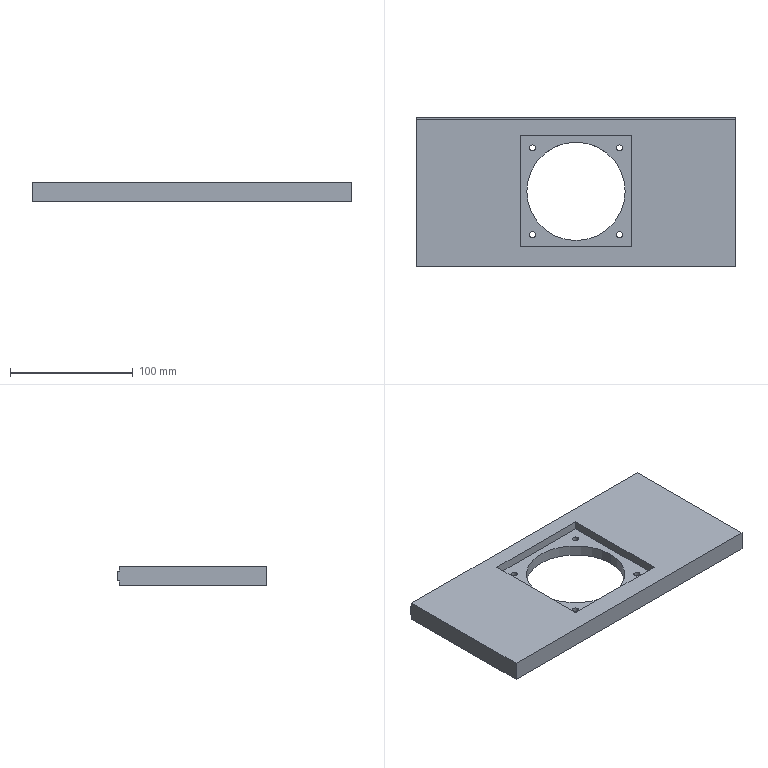Component | SolidWorks | NewTypeCurveBenderReducerPlate-DoubleWheel-2_NewTypeCurveBenderReducerPlate-DoubleWheel-1 | 1 solid | 25 faces | box 260 x 122 x 16 mm | volume 400082 mm3 | plane 15 | cylinder 10 | commonest cylinder face diameters 5 x8 80 x2
STEP:
#1=CARTESIAN_POINT('',(1.49,-3.38,7.559));
#2=VERTEX_POINT('',#1);
#3=CARTESIAN_POINT('',(1.294,-3.38,7.559));
#4=VERTEX_POINT('',#3);
#5=CARTESIAN_POINT('',(1.392,-3.38,7.559));
#6=DIRECTION('',(-0.,-0.,1.));
#7=DIRECTION('',(-1.,0.,0.));
#8=AXIS2_PLACEMENT_3D('',#5,#6,#7);
#9=CIRCLE('',#8,0.09843);
#10=EDGE_CURVE('',#2,#4,#9,.T.);
#11=ORIENTED_EDGE('',*,*,#10,.F.);
#12=CARTESIAN_POINT('',(1.49,-3.38,7.913));
#13=VERTEX_POINT('',#12);
#14=CARTESIAN_POINT('',(1.49,-3.38,8.031));
#15=DIRECTION('',(-0.,-0.,1.));
#16=VECTOR('',#15,39.37);
#17=LINE('',#14,#16);
#18=EDGE_CURVE('',#2,#13,#17,.T.);
#19=ORIENTED_EDGE('',*,*,#18,.T.);
#20=CARTESIAN_POINT('',(1.294,-3.38,7.913));
#21=VERTEX_POINT('',#20);
#22=CARTESIAN_POINT('',(1.392,-3.38,7.913));
#23=DIRECTION('',(-0.,-0.,1.));
#24=DIRECTION('',(1.,0.,0.));
#25=AXIS2_PLACEMENT_3D('',#22,#23,#24);
#26=CIRCLE('',#25,0.09843);
#27=EDGE_CURVE('',#13,#21,#26,.T.);
#28=ORIENTED_EDGE('',*,*,#27,.T.);
#29=CARTESIAN_POINT('',(1.294,-3.38,8.031));
#30=DIRECTION('',(-0.,-0.,1.));
#31=VECTOR('',#30,39.37);
#32=LINE('',#29,#31);
#33=EDGE_CURVE('',#4,#21,#32,.T.);
#34=ORIENTED_EDGE('',*,*,#33,.F.);
#35=EDGE_LOOP('',(#11,#19,#28,#34));
#36=FACE_OUTER_BOUND('',#35,.T.);
#37=CARTESIAN_POINT('',(1.392,-3.38,8.031));
#38=DIRECTION('',(-0.,-0.,1.));
#39=DIRECTION('',(-1.,0.,0.));
#40=AXIS2_PLACEMENT_3D('',#37,#38,#39);
#41=CYLINDRICAL_SURFACE('',#40,0.09843);
#42=ADVANCED_FACE('',(#36),#41,.F.);
#43=CARTESIAN_POINT('',(-1.294,-3.38,7.559));
#44=VERTEX_POINT('',#43);
#45=CARTESIAN_POINT('',(-1.49,-3.38,7.559));
#46=VERTEX_POINT('',#45);
#47=CARTESIAN_POINT('',(-1.392,-3.38,7.559));
#48=DIRECTION('',(-0.,-0.,1.));
#49=DIRECTION('',(-1.,0.,0.));
#50=AXIS2_PLACEMENT_3D('',#47,#48,#49);
#51=CIRCLE('',#50,0.09843);
#52=EDGE_CURVE('',#44,#46,#51,.T.);
#53=ORIENTED_EDGE('',*,*,#52,.F.);
#54=CARTESIAN_POINT('',(-1.294,-3.38,7.913));
#55=VERTEX_POINT('',#54);
#56=CARTESIAN_POINT('',(-1.294,-3.38,8.031));
#57=DIRECTION('',(-0.,-0.,1.));
#58=VECTOR('',#57,39.37);
#59=LINE('',#56,#58);
#60=EDGE_CURVE('',#44,#55,#59,.T.);
#61=ORIENTED_EDGE('',*,*,#60,.T.);
#62=CARTESIAN_POINT('',(-1.49,-3.38,7.913));
#63=VERTEX_POINT('',#62);
#64=CARTESIAN_POINT('',(-1.392,-3.38,7.913));
#65=DIRECTION('',(-0.,-0.,1.));
#66=DIRECTION('',(1.,0.,0.));
#67=AXIS2_PLACEMENT_3D('',#64,#65,#66);
#68=CIRCLE('',#67,0.09843);
#69=EDGE_CURVE('',#55,#63,#68,.T.);
#70=ORIENTED_EDGE('',*,*,#69,.T.);
#71=CARTESIAN_POINT('',(-1.49,-3.38,8.031));
#72=DIRECTION('',(-0.,-0.,1.));
#73=VECTOR('',#72,39.37);
#74=LINE('',#71,#73);
#75=EDGE_CURVE('',#46,#63,#74,.T.);
#76=ORIENTED_EDGE('',*,*,#75,.F.);
#77=EDGE_LOOP('',(#53,#61,#70,#76));
#78=FACE_OUTER_BOUND('',#77,.T.);
#79=CARTESIAN_POINT('',(-1.392,-3.38,8.031));
#80=DIRECTION('',(-0.,-0.,1.));
#81=DIRECTION('',(-1.,0.,0.));
#82=AXIS2_PLACEMENT_3D('',#79,#80,#81);
#83=CYLINDRICAL_SURFACE('',#82,0.09843);
#84=ADVANCED_FACE('',(#78),#83,.F.);
#85=CARTESIAN_POINT('',(-1.294,-0.5962,7.559));
#86=VERTEX_POINT('',#85);
#87=CARTESIAN_POINT('',(-1.49,-0.5962,7.559));
#88=VERTEX_POINT('',#87);
#89=CARTESIAN_POINT('',(-1.392,-0.5962,7.559));
#90=DIRECTION('',(-0.,-0.,1.));
#91=DIRECTION('',(-1.,0.,0.));
#92=AXIS2_PLACEMENT_3D('',#89,#90,#91);
#93=CIRCLE('',#92,0.09843);
#94=EDGE_CURVE('',#86,#88,#93,.T.);
#95=ORIENTED_EDGE('',*,*,#94,.F.);
#96=CARTESIAN_POINT('',(-1.294,-0.5962,7.913));
#97=VERTEX_POINT('',#96);
#98=CARTESIAN_POINT('',(-1.294,-0.5962,8.031));
#99=DIRECTION('',(-0.,-0.,1.));
#100=VECTOR('',#99,39.37);
#101=LINE('',#98,#100);
#102=EDGE_CURVE('',#86,#97,#101,.T.);
#103=ORIENTED_EDGE('',*,*,#102,.T.);
#104=CARTESIAN_POINT('',(-1.49,-0.5962,7.913));
#105=VERTEX_POINT('',#104);
#106=CARTESIAN_POINT('',(-1.392,-0.5962,7.913));
#107=DIRECTION('',(-0.,-0.,1.));
#108=DIRECTION('',(1.,0.,0.));
#109=AXIS2_PLACEMENT_3D('',#106,#107,#108);
#110=CIRCLE('',#109,0.09843);
#111=EDGE_CURVE('',#97,#105,#110,.T.);
#112=ORIENTED_EDGE('',*,*,#111,.T.);
#113=CARTESIAN_POINT('',(-1.49,-0.5962,8.031));
#114=DIRECTION('',(-0.,-0.,1.));
#115=VECTOR('',#114,39.37);
#116=LINE('',#113,#115);
#117=EDGE_CURVE('',#88,#105,#116,.T.);
#118=ORIENTED_EDGE('',*,*,#117,.F.);
#119=EDGE_LOOP('',(#95,#103,#112,#118));
#120=FACE_OUTER_BOUND('',#119,.T.);
#121=CARTESIAN_POINT('',(-1.392,-0.5962,8.031));
#122=DIRECTION('',(-0.,-0.,1.));
#123=DIRECTION('',(-1.,0.,0.));
#124=AXIS2_PLACEMENT_3D('',#121,#122,#123);
#125=CYLINDRICAL_SURFACE('',#124,0.09843);
#126=ADVANCED_FACE('',(#120),#125,.F.);
#127=CARTESIAN_POINT('',(1.49,-0.5962,7.559));
#128=VERTEX_POINT('',#127);
#129=CARTESIAN_POINT('',(1.294,-0.5962,7.559));
#130=VERTEX_POINT('',#129);
#131=CARTESIAN_POINT('',(1.392,-0.5962,7.559));
#132=DIRECTION('',(-0.,-0.,1.));
#133=DIRECTION('',(-1.,0.,0.));
#134=AXIS2_PLACEMENT_3D('',#131,#132,#133);
#135=CIRCLE('',#134,0.09843);
#136=EDGE_CURVE('',#128,#130,#135,.T.);
#137=ORIENTED_EDGE('',*,*,#136,.F.);
#138=CARTESIAN_POINT('',(1.49,-0.5962,7.913));
#139=VERTEX_POINT('',#138);
#140=CARTESIAN_POINT('',(1.49,-0.5962,8.031));
#141=DIRECTION('',(-0.,-0.,1.));
#142=VECTOR('',#141,39.37);
#143=LINE('',#140,#142);
#144=EDGE_CURVE('',#128,#139,#143,.T.);
#145=ORIENTED_EDGE('',*,*,#144,.T.);
#146=CARTESIAN_POINT('',(1.294,-0.5962,7.913));
#147=VERTEX_POINT('',#146);
#148=CARTESIAN_POINT('',(1.392,-0.5962,7.913));
#149=DIRECTION('',(-0.,-0.,1.));
#150=DIRECTION('',(1.,0.,0.));
#151=AXIS2_PLACEMENT_3D('',#148,#149,#150);
#152=CIRCLE('',#151,0.09843);
#153=EDGE_CURVE('',#139,#147,#152,.T.);
#154=ORIENTED_EDGE('',*,*,#153,.T.);
#155=CARTESIAN_POINT('',(1.294,-0.5962,8.031));
#156=DIRECTION('',(-0.,-0.,1.));
#157=VECTOR('',#156,39.37);
#158=LINE('',#155,#157);
#159=EDGE_CURVE('',#130,#147,#158,.T.);
#160=ORIENTED_EDGE('',*,*,#159,.F.);
#161=EDGE_LOOP('',(#137,#145,#154,#160));
#162=FACE_OUTER_BOUND('',#161,.T.);
#163=CARTESIAN_POINT('',(1.392,-0.5962,8.031));
#164=DIRECTION('',(-0.,-0.,1.));
#165=DIRECTION('',(-1.,0.,0.));
#166=AXIS2_PLACEMENT_3D('',#163,#164,#165);
#167=CYLINDRICAL_SURFACE('',#166,0.09843);
#168=ADVANCED_FACE('',(#162),#167,.F.);
#169=CARTESIAN_POINT('',(1.575,-1.988,7.559));
#170=VERTEX_POINT('',#169);
#171=CARTESIAN_POINT('',(-1.575,-1.988,7.559));
#172=VERTEX_POINT('',#171);
#173=CARTESIAN_POINT('',(0.,-1.988,7.559));
#174=DIRECTION('',(-0.,-0.,1.));
#175=DIRECTION('',(-1.,0.,0.));
#176=AXIS2_PLACEMENT_3D('',#173,#174,#175);
#177=CIRCLE('',#176,1.575);
#178=EDGE_CURVE('',#170,#172,#177,.T.);
#179=ORIENTED_EDGE('',*,*,#178,.F.);
#180=CARTESIAN_POINT('',(1.575,-1.988,7.913));
#181=VERTEX_POINT('',#180);
#182=CARTESIAN_POINT('',(1.575,-1.988,7.402));
#183=DIRECTION('',(-0.,-0.,1.));
#184=VECTOR('',#183,39.37);
#185=LINE('',#182,#184);
#186=EDGE_CURVE('',#170,#181,#185,.T.);
#187=ORIENTED_EDGE('',*,*,#186,.T.);
#188=CARTESIAN_POINT('',(-1.575,-1.988,7.913));
#189=VERTEX_POINT('',#188);
#190=CARTESIAN_POINT('',(0.,-1.988,7.913));
#191=DIRECTION('',(-0.,-0.,1.));
#192=DIRECTION('',(1.,0.,0.));
#193=AXIS2_PLACEMENT_3D('',#190,#191,#192);
#194=CIRCLE('',#193,1.575);
#195=EDGE_CURVE('',#181,#189,#194,.T.);
#196=ORIENTED_EDGE('',*,*,#195,.T.);
#197=CARTESIAN_POINT('',(-1.575,-1.988,7.402));
#198=DIRECTION('',(-0.,-0.,1.));
#199=VECTOR('',#198,39.37);
#200=LINE('',#197,#199);
#201=EDGE_CURVE('',#172,#189,#200,.T.);
#202=ORIENTED_EDGE('',*,*,#201,.F.);
#203=EDGE_LOOP('',(#179,#187,#196,#202));
#204=FACE_OUTER_BOUND('',#203,.T.);
#205=CARTESIAN_POINT('',(0.,-1.988,7.402));
#206=DIRECTION('',(-0.,-0.,1.));
#207=DIRECTION('',(-1.,0.,0.));
#208=AXIS2_PLACEMENT_3D('',#205,#206,#207);
#209=CYLINDRICAL_SURFACE('',#208,1.575);
#210=ADVANCED_FACE('',(#204),#209,.F.);
#211=CARTESIAN_POINT('',(-5.118,0.315,8.031));
#212=VERTEX_POINT('',#211);
#213=CARTESIAN_POINT('',(5.118,0.315,8.031));
#214=VERTEX_POINT('',#213);
#215=CARTESIAN_POINT('',(-5.118,0.315,8.031));
#216=DIRECTION('',(1.,-0.,0.));
#217=VECTOR('',#216,39.37);
#218=LINE('',#215,#217);
#219=EDGE_CURVE('',#212,#214,#218,.T.);
#220=ORIENTED_EDGE('',*,*,#219,.F.);
#221=CARTESIAN_POINT('',(-5.118,0.315,8.189));
#222=VERTEX_POINT('',#221);
#223=CARTESIAN_POINT('',(-5.118,0.315,8.189));
#224=DIRECTION('',(0.,0.,-1.));
#225=VECTOR('',#224,39.37);
#226=LINE('',#223,#225);
#227=EDGE_CURVE('',#222,#212,#226,.T.);
#228=ORIENTED_EDGE('',*,*,#227,.F.);
#229=CARTESIAN_POINT('',(5.118,0.315,8.189));
#230=VERTEX_POINT('',#229);
#231=CARTESIAN_POINT('',(5.118,0.315,8.189));
#232=DIRECTION('',(-1.,0.,-0.));
#233=VECTOR('',#232,39.37);
#234=LINE('',#231,#233);
#235=EDGE_CURVE('',#230,#222,#234,.T.);
#236=ORIENTED_EDGE('',*,*,#235,.F.);
#237=CARTESIAN_POINT('',(5.118,0.315,8.189));
#238=DIRECTION('',(0.,0.,-1.));
#239=VECTOR('',#238,39.37);
#240=LINE('',#237,#239);
#241=EDGE_CURVE('',#230,#214,#240,.T.);
#242=ORIENTED_EDGE('',*,*,#241,.T.);
#243=EDGE_LOOP('',(#220,#228,#236,#242));
#244=FACE_OUTER_BOUND('',#243,.T.);
#245=CARTESIAN_POINT('',(5.118,0.315,8.189));
#246=DIRECTION('',(-0.,-1.,-0.));
#247=DIRECTION('',(-0.,-0.,1.));
#248=AXIS2_PLACEMENT_3D('',#245,#246,#247);
#249=PLANE('',#248);
#250=ADVANCED_FACE('',(#244),#249,.F.);
#251=CARTESIAN_POINT('',(-5.118,0.315,7.559));
#252=VERTEX_POINT('',#251);
#253=CARTESIAN_POINT('',(-5.118,-4.409,7.559));
#254=VERTEX_POINT('',#253);
#255=CARTESIAN_POINT('',(-5.118,-4.409,7.559));
#256=DIRECTION('',(0.,-1.,-0.));
#257=VECTOR('',#256,39.37);
#258=LINE('',#255,#257);
#259=EDGE_CURVE('',#252,#254,#258,.T.);
#260=ORIENTED_EDGE('',*,*,#259,.T.);
#261=CARTESIAN_POINT('',(-5.118,-4.409,8.189));
#262=VERTEX_POINT('',#261);
#263=CARTESIAN_POINT('',(-5.118,-4.409,8.189));
#264=DIRECTION('',(0.,0.,-1.));
#265=VECTOR('',#264,39.37);
#266=LINE('',#263,#265);
#267=EDGE_CURVE('',#262,#254,#266,.T.);
#268=ORIENTED_EDGE('',*,*,#267,.F.);
#269=CARTESIAN_POINT('',(-5.118,-4.409,8.189));
#270=DIRECTION('',(0.,-1.,-0.));
#271=VECTOR('',#270,39.37);
#272=LINE('',#269,#271);
#273=EDGE_CURVE('',#222,#262,#272,.T.);
#274=ORIENTED_EDGE('',*,*,#273,.F.);
#275=ORIENTED_EDGE('',*,*,#227,.T.);
#276=CARTESIAN_POINT('',(-5.118,0.3937,8.031));
#277=VERTEX_POINT('',#276);
#278=CARTESIAN_POINT('',(-5.118,0.315,8.031));
#279=DIRECTION('',(-0.,-1.,-0.));
#280=VECTOR('',#279,39.37);
#281=LINE('',#278,#280);
#282=EDGE_CURVE('',#277,#212,#281,.T.);
#283=ORIENTED_EDGE('',*,*,#282,.F.);
#284=CARTESIAN_POINT('',(-5.118,0.3937,7.717));
#285=VERTEX_POINT('',#284);
#286=CARTESIAN_POINT('',(-5.118,0.3937,7.717));
#287=DIRECTION('',(-0.,-0.,1.));
#288=VECTOR('',#287,39.37);
#289=LINE('',#286,#288);
#290=EDGE_CURVE('',#285,#277,#289,.T.);
#291=ORIENTED_EDGE('',*,*,#290,.F.);
#292=CARTESIAN_POINT('',(-5.118,0.315,7.717));
#293=VERTEX_POINT('',#292);
#294=CARTESIAN_POINT('',(-5.118,0.315,7.717));
#295=DIRECTION('',(0.,1.,0.));
#296=VECTOR('',#295,39.37);
#297=LINE('',#294,#296);
#298=EDGE_CURVE('',#293,#285,#297,.T.);
#299=ORIENTED_EDGE('',*,*,#298,.F.);
#300=CARTESIAN_POINT('',(-5.118,0.315,8.189));
#301=DIRECTION('',(0.,0.,-1.));
#302=VECTOR('',#301,39.37);
#303=LINE('',#300,#302);
#304=EDGE_CURVE('',#293,#252,#303,.T.);
#305=ORIENTED_EDGE('',*,*,#304,.T.);
#306=EDGE_LOOP('',(#260,#268,#274,#275,#283,#291,#299,#305));
#307=FACE_OUTER_BOUND('',#306,.T.);
#308=CARTESIAN_POINT('',(-5.118,-4.409,8.189));
#309=DIRECTION('',(1.,0.,0.));
#310=DIRECTION('',(-0.,1.,0.));
#311=AXIS2_PLACEMENT_3D('',#308,#309,#310);
#312=PLANE('',#311);
#313=ADVANCED_FACE('',(#307),#312,.F.);
#314=CARTESIAN_POINT('',(5.118,-4.409,7.559));
#315=VERTEX_POINT('',#314);
#316=CARTESIAN_POINT('',(5.118,-4.409,7.559));
#317=DIRECTION('',(1.,-0.,0.));
#318=VECTOR('',#317,39.37);
#319=LINE('',#316,#318);
#320=EDGE_CURVE('',#254,#315,#319,.T.);
#321=ORIENTED_EDGE('',*,*,#320,.T.);
#322=CARTESIAN_POINT('',(5.118,-4.409,8.189));
#323=VERTEX_POINT('',#322);
#324=CARTESIAN_POINT('',(5.118,-4.409,8.189));
#325=DIRECTION('',(0.,0.,-1.));
#326=VECTOR('',#325,39.37);
#327=LINE('',#324,#326);
#328=EDGE_CURVE('',#323,#315,#327,.T.);
#329=ORIENTED_EDGE('',*,*,#328,.F.);
#330=CARTESIAN_POINT('',(5.118,-4.409,8.189));
#331=DIRECTION('',(1.,-0.,0.));
#332=VECTOR('',#331,39.37);
#333=LINE('',#330,#332);
#334=EDGE_CURVE('',#262,#323,#333,.T.);
#335=ORIENTED_EDGE('',*,*,#334,.F.);
#336=ORIENTED_EDGE('',*,*,#267,.T.);
#337=EDGE_LOOP('',(#321,#329,#335,#336));
#338=FACE_OUTER_BOUND('',#337,.T.);
#339=CARTESIAN_POINT('',(5.118,-4.409,8.189));
#340=DIRECTION('',(0.,1.,0.));
#341=DIRECTION('',(0.,0.,-1.));
#342=AXIS2_PLACEMENT_3D('',#339,#340,#341);
#343=PLANE('',#342);
#344=ADVANCED_FACE('',(#338),#343,.F.);
#345=CARTESIAN_POINT('',(5.118,0.315,7.559));
#346=VERTEX_POINT('',#345);
#347=CARTESIAN_POINT('',(5.118,-4.409,7.559));
#348=DIRECTION('',(-0.,1.,0.));
#349=VECTOR('',#348,39.37);
#350=LINE('',#347,#349);
#351=EDGE_CURVE('',#315,#346,#350,.T.);
#352=ORIENTED_EDGE('',*,*,#351,.T.);
#353=CARTESIAN_POINT('',(5.118,0.315,7.717));
#354=VERTEX_POINT('',#353);
#355=CARTESIAN_POINT('',(5.118,0.315,8.189));
#356=DIRECTION('',(0.,0.,-1.));
#357=VECTOR('',#356,39.37);
#358=LINE('',#355,#357);
#359=EDGE_CURVE('',#354,#346,#358,.T.);
#360=ORIENTED_EDGE('',*,*,#359,.F.);
#361=CARTESIAN_POINT('',(5.118,0.3937,7.717));
#362=VERTEX_POINT('',#361);
#363=CARTESIAN_POINT('',(5.118,0.315,7.717));
#364=DIRECTION('',(0.,1.,0.));
#365=VECTOR('',#364,39.37);
#366=LINE('',#363,#365);
#367=EDGE_CURVE('',#354,#362,#366,.T.);
#368=ORIENTED_EDGE('',*,*,#367,.T.);
#369=CARTESIAN_POINT('',(5.118,0.3937,8.031));
#370=VERTEX_POINT('',#369);
#371=CARTESIAN_POINT('',(5.118,0.3937,7.717));
#372=DIRECTION('',(-0.,-0.,1.));
#373=VECTOR('',#372,39.37);
#374=LINE('',#371,#373);
#375=EDGE_CURVE('',#362,#370,#374,.T.);
#376=ORIENTED_EDGE('',*,*,#375,.T.);
#377=CARTESIAN_POINT('',(5.118,0.315,8.031));
#378=DIRECTION('',(-0.,-1.,-0.));
#379=VECTOR('',#378,39.37);
#380=LINE('',#377,#379);
#381=EDGE_CURVE('',#370,#214,#380,.T.);
#382=ORIENTED_EDGE('',*,*,#381,.T.);
#383=ORIENTED_EDGE('',*,*,#241,.F.);
#384=CARTESIAN_POINT('',(5.118,-4.409,8.189));
#385=DIRECTION('',(-0.,1.,0.));
#386=VECTOR('',#385,39.37);
#387=LINE('',#384,#386);
#388=EDGE_CURVE('',#323,#230,#387,.T.);
#389=ORIENTED_EDGE('',*,*,#388,.F.);
#390=ORIENTED_EDGE('',*,*,#328,.T.);
#391=EDGE_LOOP('',(#352,#360,#368,#376,#382,#383,#389,#390));
#392=FACE_OUTER_BOUND('',#391,.T.);
#393=CARTESIAN_POINT('',(5.118,-4.409,8.189));
#394=DIRECTION('',(-1.,-0.,-0.));
#395=DIRECTION('',(0.,-1.,-0.));
#396=AXIS2_PLACEMENT_3D('',#393,#394,#395);
#397=PLANE('',#396);
#398=ADVANCED_FACE('',(#392),#397,.F.);
#399=ORIENTED_EDGE('',*,*,#304,.F.);
#400=CARTESIAN_POINT('',(-5.118,0.315,7.717));
#401=DIRECTION('',(1.,-0.,0.));
#402=VECTOR('',#401,39.37);
#403=LINE('',#400,#402);
#404=EDGE_CURVE('',#293,#354,#403,.T.);
#405=ORIENTED_EDGE('',*,*,#404,.T.);
#406=ORIENTED_EDGE('',*,*,#359,.T.);
#407=CARTESIAN_POINT('',(5.118,0.315,7.559));
#408=DIRECTION('',(-1.,0.,-0.));
#409=VECTOR('',#408,39.37);
#410=LINE('',#407,#409);
#411=EDGE_CURVE('',#346,#252,#410,.T.);
#412=ORIENTED_EDGE('',*,*,#411,.T.);
#413=EDGE_LOOP('',(#399,#405,#406,#412));
#414=FACE_OUTER_BOUND('',#413,.T.);
#415=CARTESIAN_POINT('',(5.118,0.315,8.189));
#416=DIRECTION('',(-0.,-1.,-0.));
#417=DIRECTION('',(-0.,-0.,1.));
#418=AXIS2_PLACEMENT_3D('',#415,#416,#417);
#419=PLANE('',#418);
#420=ADVANCED_FACE('',(#414),#419,.F.);
#421=CARTESIAN_POINT('',(1.781,-0.2067,8.189));
#422=VERTEX_POINT('',#421);
#423=CARTESIAN_POINT('',(-1.781,-0.2067,8.189));
#424=VERTEX_POINT('',#423);
#425=CARTESIAN_POINT('',(0.,-0.2067,8.189));
#426=DIRECTION('',(-1.,0.,-0.));
#427=VECTOR('',#426,39.37);
#428=LINE('',#425,#427);
#429=EDGE_CURVE('',#422,#424,#428,.T.);
#430=ORIENTED_EDGE('',*,*,#429,.F.);
#431=CARTESIAN_POINT('',(1.781,-3.77,8.189));
#432=VERTEX_POINT('',#431);
#433=CARTESIAN_POINT('',(1.781,-2.047,8.189));
#434=DIRECTION('',(0.,1.,0.));
#435=VECTOR('',#434,39.37);
#436=LINE('',#433,#435);
#437=EDGE_CURVE('',#432,#422,#436,.T.);
#438=ORIENTED_EDGE('',*,*,#437,.F.);
#439=CARTESIAN_POINT('',(-1.781,-3.77,8.189));
#440=VERTEX_POINT('',#439);
#441=CARTESIAN_POINT('',(0.,-3.77,8.189));
#442=DIRECTION('',(1.,-0.,0.));
#443=VECTOR('',#442,39.37);
#444=LINE('',#441,#443);
#445=EDGE_CURVE('',#440,#432,#444,.T.);
#446=ORIENTED_EDGE('',*,*,#445,.F.);
#447=CARTESIAN_POINT('',(-1.781,-2.047,8.189));
#448=DIRECTION('',(-0.,-1.,-0.));
#449=VECTOR('',#448,39.37);
#450=LINE('',#447,#449);
#451=EDGE_CURVE('',#424,#440,#450,.T.);
#452=ORIENTED_EDGE('',*,*,#451,.F.);
#453=EDGE_LOOP('',(#430,#438,#446,#452));
#454=FACE_BOUND('',#453,.T.);
#455=ORIENTED_EDGE('',*,*,#273,.T.);
#456=ORIENTED_EDGE('',*,*,#334,.T.);
#457=ORIENTED_EDGE('',*,*,#388,.T.);
#458=ORIENTED_EDGE('',*,*,#235,.T.);
#459=EDGE_LOOP('',(#455,#456,#457,#458));
#460=FACE_OUTER_BOUND('',#459,.T.);
#461=CARTESIAN_POINT('',(0.,-2.047,8.189));
#462=DIRECTION('',(-0.,-0.,1.));
#463=DIRECTION('',(-1.,0.,-0.));
#464=AXIS2_PLACEMENT_3D('',#461,#462,#463);
#465=PLANE('',#464);
#466=ADVANCED_FACE('',(#454,#460),#465,.T.);
#467=CARTESIAN_POINT('',(1.392,-3.38,7.559));
#468=DIRECTION('',(-0.,-0.,1.));
#469=DIRECTION('',(-1.,0.,0.));
#470=AXIS2_PLACEMENT_3D('',#467,#468,#469);
#471=CIRCLE('',#470,0.09843);
#472=EDGE_CURVE('',#4,#2,#471,.T.);
#473=ORIENTED_EDGE('',*,*,#472,.T.);
#474=ORIENTED_EDGE('',*,*,#10,.T.);
#475=EDGE_LOOP('',(#473,#474));
#476=FACE_BOUND('',#475,.T.);
#477=CARTESIAN_POINT('',(-1.392,-3.38,7.559));
#478=DIRECTION('',(-0.,-0.,1.));
#479=DIRECTION('',(-1.,0.,0.));
#480=AXIS2_PLACEMENT_3D('',#477,#478,#479);
#481=CIRCLE('',#480,0.09843);
#482=EDGE_CURVE('',#46,#44,#481,.T.);
#483=ORIENTED_EDGE('',*,*,#482,.T.);
#484=ORIENTED_EDGE('',*,*,#52,.T.);
#485=EDGE_LOOP('',(#483,#484));
#486=FACE_BOUND('',#485,.T.);
#487=CARTESIAN_POINT('',(-1.392,-0.5962,7.559));
#488=DIRECTION('',(-0.,-0.,1.));
#489=DIRECTION('',(-1.,0.,0.));
#490=AXIS2_PLACEMENT_3D('',#487,#488,#489);
#491=CIRCLE('',#490,0.09843);
#492=EDGE_CURVE('',#88,#86,#491,.T.);
#493=ORIENTED_EDGE('',*,*,#492,.T.);
#494=ORIENTED_EDGE('',*,*,#94,.T.);
#495=EDGE_LOOP('',(#493,#494));
#496=FACE_BOUND('',#495,.T.);
#497=CARTESIAN_POINT('',(1.392,-0.5962,7.559));
#498=DIRECTION('',(-0.,-0.,1.));
#499=DIRECTION('',(-1.,0.,0.));
#500=AXIS2_PLACEMENT_3D('',#497,#498,#499);
#501=CIRCLE('',#500,0.09843);
#502=EDGE_CURVE('',#130,#128,#501,.T.);
#503=ORIENTED_EDGE('',*,*,#502,.T.);
#504=ORIENTED_EDGE('',*,*,#136,.T.);
#505=EDGE_LOOP('',(#503,#504));
#506=FACE_BOUND('',#505,.T.);
#507=CARTESIAN_POINT('',(0.,-1.988,7.559));
#508=DIRECTION('',(-0.,-0.,1.));
#509=DIRECTION('',(-1.,0.,0.));
#510=AXIS2_PLACEMENT_3D('',#507,#508,#509);
#511=CIRCLE('',#510,1.575);
#512=EDGE_CURVE('',#172,#170,#511,.T.);
#513=ORIENTED_EDGE('',*,*,#512,.T.);
#514=ORIENTED_EDGE('',*,*,#178,.T.);
#515=EDGE_LOOP('',(#513,#514));
#516=FACE_BOUND('',#515,.T.);
#517=ORIENTED_EDGE('',*,*,#259,.F.);
#518=ORIENTED_EDGE('',*,*,#411,.F.);
#519=ORIENTED_EDGE('',*,*,#351,.F.);
#520=ORIENTED_EDGE('',*,*,#320,.F.);
#521=EDGE_LOOP('',(#517,#518,#519,#520));
#522=FACE_OUTER_BOUND('',#521,.T.);
#523=CARTESIAN_POINT('',(0.,-2.047,7.559));
#524=DIRECTION('',(-0.,-0.,1.));
#525=DIRECTION('',(-1.,0.,-0.));
#526=AXIS2_PLACEMENT_3D('',#523,#524,#525);
#527=PLANE('',#526);
#528=ADVANCED_FACE('',(#476,#486,#496,#506,#516,#522),#527,.F.);
#529=ORIENTED_EDGE('',*,*,#186,.F.);
#530=ORIENTED_EDGE('',*,*,#512,.F.);
#531=ORIENTED_EDGE('',*,*,#201,.T.);
#532=CARTESIAN_POINT('',(0.,-1.988,7.913));
#533=DIRECTION('',(-0.,-0.,1.));
#534=DIRECTION('',(1.,0.,0.));
#535=AXIS2_PLACEMENT_3D('',#532,#533,#534);
#536=CIRCLE('',#535,1.575);
#537=EDGE_CURVE('',#189,#181,#536,.T.);
#538=ORIENTED_EDGE('',*,*,#537,.T.);
#539=EDGE_LOOP('',(#529,#530,#531,#538));
#540=FACE_OUTER_BOUND('',#539,.T.);
#541=CARTESIAN_POINT('',(0.,-1.988,7.402));
#542=DIRECTION('',(-0.,-0.,1.));
#543=DIRECTION('',(-1.,0.,0.));
#544=AXIS2_PLACEMENT_3D('',#541,#542,#543);
#545=CYLINDRICAL_SURFACE('',#544,1.575);
#546=ADVANCED_FACE('',(#540),#545,.F.);
#547=ORIENTED_EDGE('',*,*,#144,.F.);
#548=ORIENTED_EDGE('',*,*,#502,.F.);
#549=ORIENTED_EDGE('',*,*,#159,.T.);
#550=CARTESIAN_POINT('',(1.392,-0.5962,7.913));
#551=DIRECTION('',(-0.,-0.,1.));
#552=DIRECTION('',(1.,0.,0.));
#553=AXIS2_PLACEMENT_3D('',#550,#551,#552);
#554=CIRCLE('',#553,0.09843);
#555=EDGE_CURVE('',#147,#139,#554,.T.);
#556=ORIENTED_EDGE('',*,*,#555,.T.);
#557=EDGE_LOOP('',(#547,#548,#549,#556));
#558=FACE_OUTER_BOUND('',#557,.T.);
#559=CARTESIAN_POINT('',(1.392,-0.5962,8.031));
#560=DIRECTION('',(-0.,-0.,1.));
#561=DIRECTION('',(-1.,0.,0.));
#562=AXIS2_PLACEMENT_3D('',#559,#560,#561);
#563=CYLINDRICAL_SURFACE('',#562,0.09843);
#564=ADVANCED_FACE('',(#558),#563,.F.);
#565=ORIENTED_EDGE('',*,*,#102,.F.);
#566=ORIENTED_EDGE('',*,*,#492,.F.);
#567=ORIENTED_EDGE('',*,*,#117,.T.);
#568=CARTESIAN_POINT('',(-1.392,-0.5962,7.913));
#569=DIRECTION('',(-0.,-0.,1.));
#570=DIRECTION('',(1.,0.,0.));
#571=AXIS2_PLACEMENT_3D('',#568,#569,#570);
#572=CIRCLE('',#571,0.09843);
#573=EDGE_CURVE('',#105,#97,#572,.T.);
#574=ORIENTED_EDGE('',*,*,#573,.T.);
#575=EDGE_LOOP('',(#565,#566,#567,#574));
#576=FACE_OUTER_BOUND('',#575,.T.);
#577=CARTESIAN_POINT('',(-1.392,-0.5962,8.031));
#578=DIRECTION('',(-0.,-0.,1.));
#579=DIRECTION('',(-1.,0.,0.));
#580=AXIS2_PLACEMENT_3D('',#577,#578,#579);
#581=CYLINDRICAL_SURFACE('',#580,0.09843);
#582=ADVANCED_FACE('',(#576),#581,.F.);
#583=ORIENTED_EDGE('',*,*,#60,.F.);
#584=ORIENTED_EDGE('',*,*,#482,.F.);
#585=ORIENTED_EDGE('',*,*,#75,.T.);
#586=CARTESIAN_POINT('',(-1.392,-3.38,7.913));
#587=DIRECTION('',(-0.,-0.,1.));
#588=DIRECTION('',(1.,0.,0.));
#589=AXIS2_PLACEMENT_3D('',#586,#587,#588);
#590=CIRCLE('',#589,0.09843);
#591=EDGE_CURVE('',#63,#55,#590,.T.);
#592=ORIENTED_EDGE('',*,*,#591,.T.);
#593=EDGE_LOOP('',(#583,#584,#585,#592));
#594=FACE_OUTER_BOUND('',#593,.T.);
#595=CARTESIAN_POINT('',(-1.392,-3.38,8.031));
#596=DIRECTION('',(-0.,-0.,1.));
#597=DIRECTION('',(-1.,0.,0.));
#598=AXIS2_PLACEMENT_3D('',#595,#596,#597);
#599=CYLINDRICAL_SURFACE('',#598,0.09843);
#600=ADVANCED_FACE('',(#594),#599,.F.);
#601=ORIENTED_EDGE('',*,*,#18,.F.);
#602=ORIENTED_EDGE('',*,*,#472,.F.);
#603=ORIENTED_EDGE('',*,*,#33,.T.);
#604=CARTESIAN_POINT('',(1.392,-3.38,7.913));
#605=DIRECTION('',(-0.,-0.,1.));
#606=DIRECTION('',(1.,0.,0.));
#607=AXIS2_PLACEMENT_3D('',#604,#605,#606);
#608=CIRCLE('',#607,0.09843);
#609=EDGE_CURVE('',#21,#13,#608,.T.);
#610=ORIENTED_EDGE('',*,*,#609,.T.);
#611=EDGE_LOOP('',(#601,#602,#603,#610));
#612=FACE_OUTER_BOUND('',#611,.T.);
#613=CARTESIAN_POINT('',(1.392,-3.38,8.031));
#614=DIRECTION('',(-0.,-0.,1.));
#615=DIRECTION('',(-1.,0.,0.));
#616=AXIS2_PLACEMENT_3D('',#613,#614,#615);
#617=CYLINDRICAL_SURFACE('',#616,0.09843);
#618=ADVANCED_FACE('',(#612),#617,.F.);
#619=ORIENTED_EDGE('',*,*,#367,.F.);
#620=ORIENTED_EDGE('',*,*,#404,.F.);
#621=ORIENTED_EDGE('',*,*,#298,.T.);
#622=CARTESIAN_POINT('',(-5.118,0.3937,7.717));
#623=DIRECTION('',(1.,-0.,0.));
#624=VECTOR('',#623,39.37);
#625=LINE('',#622,#624);
#626=EDGE_CURVE('',#285,#362,#625,.T.);
#627=ORIENTED_EDGE('',*,*,#626,.T.);
#628=EDGE_LOOP('',(#619,#620,#621,#627));
#629=FACE_OUTER_BOUND('',#628,.T.);
#630=CARTESIAN_POINT('',(-5.118,0.315,7.717));
#631=DIRECTION('',(0.,0.,-1.));
#632=DIRECTION('',(1.,-0.,0.));
#633=AXIS2_PLACEMENT_3D('',#630,#631,#632);
#634=PLANE('',#633);
#635=ADVANCED_FACE('',(#629),#634,.T.);
#636=ORIENTED_EDGE('',*,*,#381,.F.);
#637=CARTESIAN_POINT('',(-5.118,0.3937,8.031));
#638=DIRECTION('',(1.,-0.,0.));
#639=VECTOR('',#638,39.37);
#640=LINE('',#637,#639);
#641=EDGE_CURVE('',#277,#370,#640,.T.);
#642=ORIENTED_EDGE('',*,*,#641,.F.);
#643=ORIENTED_EDGE('',*,*,#282,.T.);
#644=ORIENTED_EDGE('',*,*,#219,.T.);
#645=EDGE_LOOP('',(#636,#642,#643,#644));
#646=FACE_OUTER_BOUND('',#645,.T.);
#647=CARTESIAN_POINT('',(-5.118,0.315,8.031));
#648=DIRECTION('',(-0.,-0.,1.));
#649=DIRECTION('',(0.,1.,0.));
#650=AXIS2_PLACEMENT_3D('',#647,#648,#649);
#651=PLANE('',#650);
#652=ADVANCED_FACE('',(#646),#651,.T.);
#653=ORIENTED_EDGE('',*,*,#375,.F.);
#654=ORIENTED_EDGE('',*,*,#626,.F.);
#655=ORIENTED_EDGE('',*,*,#290,.T.);
#656=ORIENTED_EDGE('',*,*,#641,.T.);
#657=EDGE_LOOP('',(#653,#654,#655,#656));
#658=FACE_OUTER_BOUND('',#657,.T.);
#659=CARTESIAN_POINT('',(-5.118,0.3937,7.717));
#660=DIRECTION('',(0.,1.,0.));
#661=DIRECTION('',(0.,0.,-1.));
#662=AXIS2_PLACEMENT_3D('',#659,#660,#661);
#663=PLANE('',#662);
#664=ADVANCED_FACE('',(#658),#663,.T.);
#665=ORIENTED_EDGE('',*,*,#555,.F.);
#666=ORIENTED_EDGE('',*,*,#153,.F.);
#667=EDGE_LOOP('',(#665,#666));
#668=FACE_BOUND('',#667,.T.);
#669=ORIENTED_EDGE('',*,*,#591,.F.);
#670=ORIENTED_EDGE('',*,*,#69,.F.);
#671=EDGE_LOOP('',(#669,#670));
#672=FACE_BOUND('',#671,.T.);
#673=CARTESIAN_POINT('',(-1.781,-0.2067,7.913));
#674=VERTEX_POINT('',#673);
#675=CARTESIAN_POINT('',(-1.781,-3.77,7.913));
#676=VERTEX_POINT('',#675);
#677=CARTESIAN_POINT('',(-1.781,-1.988,7.913));
#678=DIRECTION('',(-0.,-1.,-0.));
#679=VECTOR('',#678,39.37);
#680=LINE('',#677,#679);
#681=EDGE_CURVE('',#674,#676,#680,.T.);
#682=ORIENTED_EDGE('',*,*,#681,.T.);
#683=CARTESIAN_POINT('',(1.781,-3.77,7.913));
#684=VERTEX_POINT('',#683);
#685=CARTESIAN_POINT('',(0.,-3.77,7.913));
#686=DIRECTION('',(1.,-0.,0.));
#687=VECTOR('',#686,39.37);
#688=LINE('',#685,#687);
#689=EDGE_CURVE('',#676,#684,#688,.T.);
#690=ORIENTED_EDGE('',*,*,#689,.T.);
#691=CARTESIAN_POINT('',(1.781,-0.2067,7.913));
#692=VERTEX_POINT('',#691);
#693=CARTESIAN_POINT('',(1.781,-1.988,7.913));
#694=DIRECTION('',(0.,1.,0.));
#695=VECTOR('',#694,39.37);
#696=LINE('',#693,#695);
#697=EDGE_CURVE('',#684,#692,#696,.T.);
#698=ORIENTED_EDGE('',*,*,#697,.T.);
#699=CARTESIAN_POINT('',(0.,-0.2067,7.913));
#700=DIRECTION('',(-1.,0.,-0.));
#701=VECTOR('',#700,39.37);
#702=LINE('',#699,#701);
#703=EDGE_CURVE('',#692,#674,#702,.T.);
#704=ORIENTED_EDGE('',*,*,#703,.T.);
#705=EDGE_LOOP('',(#682,#690,#698,#704));
#706=FACE_OUTER_BOUND('',#705,.T.);
#707=ORIENTED_EDGE('',*,*,#609,.F.);
#708=ORIENTED_EDGE('',*,*,#27,.F.);
#709=EDGE_LOOP('',(#707,#708));
#710=FACE_BOUND('',#709,.T.);
#711=ORIENTED_EDGE('',*,*,#573,.F.);
#712=ORIENTED_EDGE('',*,*,#111,.F.);
#713=EDGE_LOOP('',(#711,#712));
#714=FACE_BOUND('',#713,.T.);
#715=ORIENTED_EDGE('',*,*,#537,.F.);
#716=ORIENTED_EDGE('',*,*,#195,.F.);
#717=EDGE_LOOP('',(#715,#716));
#718=FACE_BOUND('',#717,.T.);
#719=CARTESIAN_POINT('',(0.,-1.988,7.913));
#720=DIRECTION('',(0.,0.,-1.));
#721=DIRECTION('',(1.,-0.,0.));
#722=AXIS2_PLACEMENT_3D('',#719,#720,#721);
#723=PLANE('',#722);
#724=ADVANCED_FACE('',(#668,#672,#706,#710,#714,#718),#723,.F.);
#725=ORIENTED_EDGE('',*,*,#429,.T.);
#726=CARTESIAN_POINT('',(-1.781,-0.2067,7.913));
#727=DIRECTION('',(-0.,-0.,1.));
#728=VECTOR('',#727,39.37);
#729=LINE('',#726,#728);
#730=EDGE_CURVE('',#674,#424,#729,.T.);
#731=ORIENTED_EDGE('',*,*,#730,.F.);
#732=ORIENTED_EDGE('',*,*,#703,.F.);
#733=CARTESIAN_POINT('',(1.781,-0.2067,7.913));
#734=DIRECTION('',(-0.,-0.,1.));
#735=VECTOR('',#734,39.37);
#736=LINE('',#733,#735);
#737=EDGE_CURVE('',#692,#422,#736,.T.);
#738=ORIENTED_EDGE('',*,*,#737,.T.);
#739=EDGE_LOOP('',(#725,#731,#732,#738));
#740=FACE_OUTER_BOUND('',#739,.T.);
#741=CARTESIAN_POINT('',(0.,-0.2067,7.913));
#742=DIRECTION('',(0.,1.,0.));
#743=DIRECTION('',(0.,0.,-1.));
#744=AXIS2_PLACEMENT_3D('',#741,#742,#743);
#745=PLANE('',#744);
#746=ADVANCED_FACE('',(#740),#745,.F.);
#747=ORIENTED_EDGE('',*,*,#437,.T.);
#748=ORIENTED_EDGE('',*,*,#737,.F.);
#749=ORIENTED_EDGE('',*,*,#697,.F.);
#750=CARTESIAN_POINT('',(1.781,-3.77,7.913));
#751=DIRECTION('',(-0.,-0.,1.));
#752=VECTOR('',#751,39.37);
#753=LINE('',#750,#752);
#754=EDGE_CURVE('',#684,#432,#753,.T.);
#755=ORIENTED_EDGE('',*,*,#754,.T.);
#756=EDGE_LOOP('',(#747,#748,#749,#755));
#757=FACE_OUTER_BOUND('',#756,.T.);
#758=CARTESIAN_POINT('',(1.781,-1.988,7.913));
#759=DIRECTION('',(1.,-0.,0.));
#760=DIRECTION('',(-0.,-0.,1.));
#761=AXIS2_PLACEMENT_3D('',#758,#759,#760);
#762=PLANE('',#761);
#763=ADVANCED_FACE('',(#757),#762,.F.);
#764=ORIENTED_EDGE('',*,*,#445,.T.);
#765=ORIENTED_EDGE('',*,*,#754,.F.);
#766=ORIENTED_EDGE('',*,*,#689,.F.);
#767=CARTESIAN_POINT('',(-1.781,-3.77,7.913));
#768=DIRECTION('',(-0.,-0.,1.));
#769=VECTOR('',#768,39.37);
#770=LINE('',#767,#769);
#771=EDGE_CURVE('',#676,#440,#770,.T.);
#772=ORIENTED_EDGE('',*,*,#771,.T.);
#773=EDGE_LOOP('',(#764,#765,#766,#772));
#774=FACE_OUTER_BOUND('',#773,.T.);
#775=CARTESIAN_POINT('',(0.,-3.77,7.913));
#776=DIRECTION('',(-0.,-1.,-0.));
#777=DIRECTION('',(-0.,-0.,1.));
#778=AXIS2_PLACEMENT_3D('',#775,#776,#777);
#779=PLANE('',#778);
#780=ADVANCED_FACE('',(#774),#779,.F.);
#781=ORIENTED_EDGE('',*,*,#451,.T.);
#782=ORIENTED_EDGE('',*,*,#771,.F.);
#783=ORIENTED_EDGE('',*,*,#681,.F.);
#784=ORIENTED_EDGE('',*,*,#730,.T.);
#785=EDGE_LOOP('',(#781,#782,#783,#784));
#786=FACE_OUTER_BOUND('',#785,.T.);
#787=CARTESIAN_POINT('',(-1.781,-1.988,7.913));
#788=DIRECTION('',(-1.,0.,-0.));
#789=DIRECTION('',(0.,0.,-1.));
#790=AXIS2_PLACEMENT_3D('',#787,#788,#789);
#791=PLANE('',#790);
#792=ADVANCED_FACE('',(#786),#791,.F.);
#793=CLOSED_SHELL('',(#42,#84,#126,#168,#210,#250,#313,#344,#398,#420,#466,#528,#546,#564,#582,#600,#618,#635,#652,#664,#724,#746,#763,#780,#792));
#794=MANIFOLD_SOLID_BREP('',#793);
#795=CARTESIAN_POINT('',(0.,0.,0.));
#796=DIRECTION('',(0.,0.,1.));
#797=DIRECTION('',(1.,0.,0.));
#798=AXIS2_PLACEMENT_3D('',#795,#796,#797);
#799=(LENGTH_UNIT()NAMED_UNIT(*)SI_UNIT($,.METRE.));
#800=LENGTH_MEASURE_WITH_UNIT(LENGTH_MEASURE(0.0254),#799);
#801=DIMENSIONAL_EXPONENTS(1.,0.,0.,0.,0.,0.,0.);
#802=(CONVERSION_BASED_UNIT('',#800)LENGTH_UNIT()NAMED_UNIT(#801));
#803=UNCERTAINTY_MEASURE_WITH_UNIT(LENGTH_MEASURE(0.00001),#802,'','');
#804=(NAMED_UNIT(*)PLANE_ANGLE_UNIT()SI_UNIT($,.RADIAN.));
#805=(NAMED_UNIT(*)SI_UNIT($,.STERADIAN.)SOLID_ANGLE_UNIT());
#806=(GEOMETRIC_REPRESENTATION_CONTEXT(3)GLOBAL_UNCERTAINTY_ASSIGNED_CONTEXT((#803))GLOBAL_UNIT_ASSIGNED_CONTEXT((#802,#804,#805))REPRESENTATION_CONTEXT('',''));
#807=ADVANCED_BREP_SHAPE_REPRESENTATION('',(#794,#798),#806);
#808=COLOUR_RGB('',0.7922,0.8196,0.9333);
#809=FILL_AREA_STYLE_COLOUR('',#808);
#810=FILL_AREA_STYLE('',(#809));
#811=SURFACE_STYLE_FILL_AREA(#810);
#812=SURFACE_SIDE_STYLE('',(#811));
#813=SURFACE_STYLE_USAGE(.BOTH.,#812);
#814=PRESENTATION_STYLE_ASSIGNMENT((#813));
#815=STYLED_ITEM('',(#814),#794);
#816=(LENGTH_UNIT()NAMED_UNIT(*)SI_UNIT($,.METRE.));
#817=LENGTH_MEASURE_WITH_UNIT(LENGTH_MEASURE(0.0254),#816);
#818=DIMENSIONAL_EXPONENTS(1.,0.,0.,0.,0.,0.,0.);
#819=(CONVERSION_BASED_UNIT('',#817)LENGTH_UNIT()NAMED_UNIT(#818));
#820=UNCERTAINTY_MEASURE_WITH_UNIT(LENGTH_MEASURE(0.00001),#819,'','');
#821=(NAMED_UNIT(*)PLANE_ANGLE_UNIT()SI_UNIT($,.RADIAN.));
#822=(NAMED_UNIT(*)SI_UNIT($,.STERADIAN.)SOLID_ANGLE_UNIT());
#823=(GEOMETRIC_REPRESENTATION_CONTEXT(3)GLOBAL_UNCERTAINTY_ASSIGNED_CONTEXT((#820))GLOBAL_UNIT_ASSIGNED_CONTEXT((#819,#821,#822))REPRESENTATION_CONTEXT('',''));
#824=MECHANICAL_DESIGN_GEOMETRIC_PRESENTATION_REPRESENTATION('',(#815),#823);
#825=PRESENTATION_LAYER_ASSIGNMENT('','',(#815));